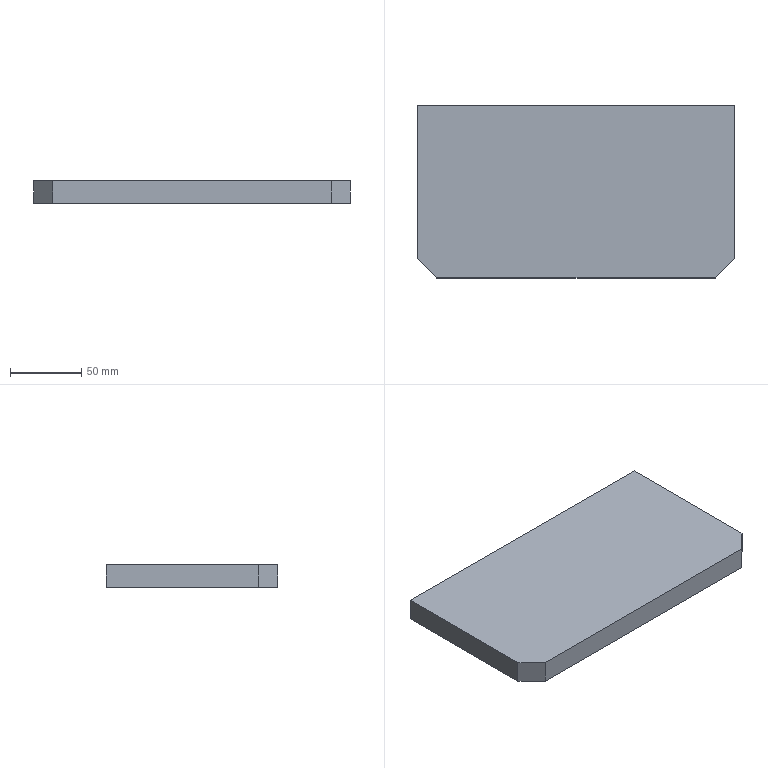Component | SolidWorks | WeldedI-beam-1_250I-beamStiffener-1 | 1 solid | 8 faces | box 222 x 120.5 x 16 mm | volume 425100 mm3 | plane 8 | material Plain Carbon Steel
STEP:
#1=COLOUR_RGB('',0.7922,0.8196,0.9333);
#2=FILL_AREA_STYLE_COLOUR('',#1);
#3=FILL_AREA_STYLE('',(#2));
#4=SURFACE_STYLE_FILL_AREA(#3);
#5=SURFACE_SIDE_STYLE('',(#4));
#6=SURFACE_STYLE_USAGE(.BOTH.,#5);
#7=PRESENTATION_STYLE_ASSIGNMENT((#6));
#8=CARTESIAN_POINT('',(-255.255,115.423,245.041));
#9=VERTEX_POINT('',#8);
#10=CARTESIAN_POINT('',(-255.255,111.21,245.041));
#11=VERTEX_POINT('',#10);
#12=CARTESIAN_POINT('',(-255.255,115.423,245.041));
#13=DIRECTION('',(0.,-1.,-0.));
#14=VECTOR('',#13,39.37);
#15=LINE('',#12,#14);
#16=EDGE_CURVE('',#9,#11,#15,.T.);
#17=ORIENTED_EDGE('',*,*,#16,.F.);
#18=CARTESIAN_POINT('',(-255.255,115.423,244.411));
#19=VERTEX_POINT('',#18);
#20=CARTESIAN_POINT('',(-255.255,115.423,244.411));
#21=DIRECTION('',(0.,-0.,1.));
#22=VECTOR('',#21,39.37);
#23=LINE('',#20,#22);
#24=EDGE_CURVE('',#19,#9,#23,.T.);
#25=ORIENTED_EDGE('',*,*,#24,.F.);
#26=CARTESIAN_POINT('',(-255.255,111.21,244.411));
#27=VERTEX_POINT('',#26);
#28=CARTESIAN_POINT('',(-255.255,115.423,244.411));
#29=DIRECTION('',(0.,-1.,-0.));
#30=VECTOR('',#29,39.37);
#31=LINE('',#28,#30);
#32=EDGE_CURVE('',#19,#27,#31,.T.);
#33=ORIENTED_EDGE('',*,*,#32,.T.);
#34=CARTESIAN_POINT('',(-255.255,111.21,244.411));
#35=DIRECTION('',(0.,-0.,1.));
#36=VECTOR('',#35,39.37);
#37=LINE('',#34,#36);
#38=EDGE_CURVE('',#27,#11,#37,.T.);
#39=ORIENTED_EDGE('',*,*,#38,.T.);
#40=EDGE_LOOP('',(#17,#25,#33,#39));
#41=FACE_OUTER_BOUND('',#40,.T.);
#42=CARTESIAN_POINT('',(-255.255,115.423,244.411));
#43=DIRECTION('',(-1.,-0.,-0.));
#44=DIRECTION('',(0.,-1.,-0.));
#45=AXIS2_PLACEMENT_3D('',#42,#43,#44);
#46=PLANE('',#45);
#47=ADVANCED_FACE('',(#41),#46,.T.);
#48=CARTESIAN_POINT('',(-246.514,115.423,245.041));
#49=VERTEX_POINT('',#48);
#50=CARTESIAN_POINT('',(-255.255,115.423,245.041));
#51=DIRECTION('',(-1.,0.,0.));
#52=VECTOR('',#51,39.37);
#53=LINE('',#50,#52);
#54=EDGE_CURVE('',#49,#9,#53,.T.);
#55=ORIENTED_EDGE('',*,*,#54,.F.);
#56=CARTESIAN_POINT('',(-246.514,115.423,244.411));
#57=VERTEX_POINT('',#56);
#58=CARTESIAN_POINT('',(-246.514,115.423,244.411));
#59=DIRECTION('',(0.,-0.,1.));
#60=VECTOR('',#59,39.37);
#61=LINE('',#58,#60);
#62=EDGE_CURVE('',#57,#49,#61,.T.);
#63=ORIENTED_EDGE('',*,*,#62,.F.);
#64=CARTESIAN_POINT('',(-255.255,115.423,244.411));
#65=DIRECTION('',(-1.,0.,0.));
#66=VECTOR('',#65,39.37);
#67=LINE('',#64,#66);
#68=EDGE_CURVE('',#57,#19,#67,.T.);
#69=ORIENTED_EDGE('',*,*,#68,.T.);
#70=ORIENTED_EDGE('',*,*,#24,.T.);
#71=EDGE_LOOP('',(#55,#63,#69,#70));
#72=FACE_OUTER_BOUND('',#71,.T.);
#73=CARTESIAN_POINT('',(-255.255,115.423,244.411));
#74=DIRECTION('',(0.,1.,0.));
#75=DIRECTION('',(-1.,0.,0.));
#76=AXIS2_PLACEMENT_3D('',#73,#74,#75);
#77=PLANE('',#76);
#78=ADVANCED_FACE('',(#72),#77,.T.);
#79=CARTESIAN_POINT('',(-246.514,111.21,245.041));
#80=VERTEX_POINT('',#79);
#81=CARTESIAN_POINT('',(-246.514,115.423,245.041));
#82=DIRECTION('',(0.,1.,0.));
#83=VECTOR('',#82,39.37);
#84=LINE('',#81,#83);
#85=EDGE_CURVE('',#80,#49,#84,.T.);
#86=ORIENTED_EDGE('',*,*,#85,.F.);
#87=CARTESIAN_POINT('',(-246.514,111.21,244.411));
#88=VERTEX_POINT('',#87);
#89=CARTESIAN_POINT('',(-246.514,111.21,244.411));
#90=DIRECTION('',(0.,-0.,1.));
#91=VECTOR('',#90,39.37);
#92=LINE('',#89,#91);
#93=EDGE_CURVE('',#88,#80,#92,.T.);
#94=ORIENTED_EDGE('',*,*,#93,.F.);
#95=CARTESIAN_POINT('',(-246.514,115.423,244.411));
#96=DIRECTION('',(0.,1.,0.));
#97=VECTOR('',#96,39.37);
#98=LINE('',#95,#97);
#99=EDGE_CURVE('',#88,#57,#98,.T.);
#100=ORIENTED_EDGE('',*,*,#99,.T.);
#101=ORIENTED_EDGE('',*,*,#62,.T.);
#102=EDGE_LOOP('',(#86,#94,#100,#101));
#103=FACE_OUTER_BOUND('',#102,.T.);
#104=CARTESIAN_POINT('',(-246.514,115.423,244.411));
#105=DIRECTION('',(1.,-0.,-0.));
#106=DIRECTION('',(0.,1.,0.));
#107=AXIS2_PLACEMENT_3D('',#104,#105,#106);
#108=PLANE('',#107);
#109=ADVANCED_FACE('',(#103),#108,.T.);
#110=CARTESIAN_POINT('',(-247.046,110.678,245.041));
#111=VERTEX_POINT('',#110);
#112=CARTESIAN_POINT('',(-247.046,110.678,245.041));
#113=DIRECTION('',(0.7071,0.7071,0.));
#114=VECTOR('',#113,39.37);
#115=LINE('',#112,#114);
#116=EDGE_CURVE('',#111,#80,#115,.T.);
#117=ORIENTED_EDGE('',*,*,#116,.F.);
#118=CARTESIAN_POINT('',(-247.046,110.678,244.411));
#119=VERTEX_POINT('',#118);
#120=CARTESIAN_POINT('',(-247.046,110.678,244.411));
#121=DIRECTION('',(0.,-0.,1.));
#122=VECTOR('',#121,39.37);
#123=LINE('',#120,#122);
#124=EDGE_CURVE('',#119,#111,#123,.T.);
#125=ORIENTED_EDGE('',*,*,#124,.F.);
#126=CARTESIAN_POINT('',(-247.046,110.678,244.411));
#127=DIRECTION('',(0.7071,0.7071,0.));
#128=VECTOR('',#127,39.37);
#129=LINE('',#126,#128);
#130=EDGE_CURVE('',#119,#88,#129,.T.);
#131=ORIENTED_EDGE('',*,*,#130,.T.);
#132=ORIENTED_EDGE('',*,*,#93,.T.);
#133=EDGE_LOOP('',(#117,#125,#131,#132));
#134=FACE_OUTER_BOUND('',#133,.T.);
#135=CARTESIAN_POINT('',(-247.046,110.678,244.411));
#136=DIRECTION('',(0.7071,-0.7071,-0.));
#137=DIRECTION('',(0.7071,0.7071,0.));
#138=AXIS2_PLACEMENT_3D('',#135,#136,#137);
#139=PLANE('',#138);
#140=ADVANCED_FACE('',(#134),#139,.T.);
#141=CARTESIAN_POINT('',(-254.723,110.678,245.041));
#142=VERTEX_POINT('',#141);
#143=CARTESIAN_POINT('',(-254.723,110.678,245.041));
#144=DIRECTION('',(1.,0.,0.));
#145=VECTOR('',#144,39.37);
#146=LINE('',#143,#145);
#147=EDGE_CURVE('',#142,#111,#146,.T.);
#148=ORIENTED_EDGE('',*,*,#147,.F.);
#149=CARTESIAN_POINT('',(-254.723,110.678,244.411));
#150=VERTEX_POINT('',#149);
#151=CARTESIAN_POINT('',(-254.723,110.678,244.411));
#152=DIRECTION('',(0.,-0.,1.));
#153=VECTOR('',#152,39.37);
#154=LINE('',#151,#153);
#155=EDGE_CURVE('',#150,#142,#154,.T.);
#156=ORIENTED_EDGE('',*,*,#155,.F.);
#157=CARTESIAN_POINT('',(-254.723,110.678,244.411));
#158=DIRECTION('',(1.,0.,0.));
#159=VECTOR('',#158,39.37);
#160=LINE('',#157,#159);
#161=EDGE_CURVE('',#150,#119,#160,.T.);
#162=ORIENTED_EDGE('',*,*,#161,.T.);
#163=ORIENTED_EDGE('',*,*,#124,.T.);
#164=EDGE_LOOP('',(#148,#156,#162,#163));
#165=FACE_OUTER_BOUND('',#164,.T.);
#166=CARTESIAN_POINT('',(-254.723,110.678,244.411));
#167=DIRECTION('',(0.,-1.,-0.));
#168=DIRECTION('',(1.,0.,0.));
#169=AXIS2_PLACEMENT_3D('',#166,#167,#168);
#170=PLANE('',#169);
#171=ADVANCED_FACE('',(#165),#170,.T.);
#172=CARTESIAN_POINT('',(-255.255,111.21,245.041));
#173=DIRECTION('',(0.7071,-0.7071,-0.));
#174=VECTOR('',#173,39.37);
#175=LINE('',#172,#174);
#176=EDGE_CURVE('',#11,#142,#175,.T.);
#177=ORIENTED_EDGE('',*,*,#176,.F.);
#178=ORIENTED_EDGE('',*,*,#38,.F.);
#179=CARTESIAN_POINT('',(-255.255,111.21,244.411));
#180=DIRECTION('',(0.7071,-0.7071,-0.));
#181=VECTOR('',#180,39.37);
#182=LINE('',#179,#181);
#183=EDGE_CURVE('',#27,#150,#182,.T.);
#184=ORIENTED_EDGE('',*,*,#183,.T.);
#185=ORIENTED_EDGE('',*,*,#155,.T.);
#186=EDGE_LOOP('',(#177,#178,#184,#185));
#187=FACE_OUTER_BOUND('',#186,.T.);
#188=CARTESIAN_POINT('',(-255.255,111.21,244.411));
#189=DIRECTION('',(-0.7071,-0.7071,-0.));
#190=DIRECTION('',(0.7071,-0.7071,-0.));
#191=AXIS2_PLACEMENT_3D('',#188,#189,#190);
#192=PLANE('',#191);
#193=ADVANCED_FACE('',(#187),#192,.T.);
#194=ORIENTED_EDGE('',*,*,#32,.F.);
#195=ORIENTED_EDGE('',*,*,#68,.F.);
#196=ORIENTED_EDGE('',*,*,#99,.F.);
#197=ORIENTED_EDGE('',*,*,#130,.F.);
#198=ORIENTED_EDGE('',*,*,#161,.F.);
#199=ORIENTED_EDGE('',*,*,#183,.F.);
#200=EDGE_LOOP('',(#194,#195,#196,#197,#198,#199));
#201=FACE_OUTER_BOUND('',#200,.T.);
#202=CARTESIAN_POINT('',(-255.255,115.423,244.411));
#203=DIRECTION('',(0.,-0.,1.));
#204=DIRECTION('',(0.,-1.,-0.));
#205=AXIS2_PLACEMENT_3D('',#202,#203,#204);
#206=PLANE('',#205);
#207=ADVANCED_FACE('',(#201),#206,.F.);
#208=ORIENTED_EDGE('',*,*,#16,.T.);
#209=ORIENTED_EDGE('',*,*,#176,.T.);
#210=ORIENTED_EDGE('',*,*,#147,.T.);
#211=ORIENTED_EDGE('',*,*,#116,.T.);
#212=ORIENTED_EDGE('',*,*,#85,.T.);
#213=ORIENTED_EDGE('',*,*,#54,.T.);
#214=EDGE_LOOP('',(#208,#209,#210,#211,#212,#213));
#215=FACE_OUTER_BOUND('',#214,.T.);
#216=CARTESIAN_POINT('',(-255.255,115.423,245.041));
#217=DIRECTION('',(0.,-0.,1.));
#218=DIRECTION('',(0.,-1.,-0.));
#219=AXIS2_PLACEMENT_3D('',#216,#217,#218);
#220=PLANE('',#219);
#221=ADVANCED_FACE('',(#215),#220,.T.);
#222=CLOSED_SHELL('',(#47,#78,#109,#140,#171,#193,#207,#221));
#223=MANIFOLD_SOLID_BREP('',#222);
#224=STYLED_ITEM('',(#7),#223);
#225=PRESENTATION_LAYER_ASSIGNMENT('','',(#224));
#226=(LENGTH_UNIT()NAMED_UNIT(*)SI_UNIT($,.METRE.));
#227=LENGTH_MEASURE_WITH_UNIT(LENGTH_MEASURE(0.0254),#226);
#228=DIMENSIONAL_EXPONENTS(1.,0.,0.,0.,0.,0.,0.);
#229=(CONVERSION_BASED_UNIT('',#227)LENGTH_UNIT()NAMED_UNIT(#228));
#230=UNCERTAINTY_MEASURE_WITH_UNIT(LENGTH_MEASURE(0.00001),#229,'','');
#231=(NAMED_UNIT(*)PLANE_ANGLE_UNIT()SI_UNIT($,.RADIAN.));
#232=(NAMED_UNIT(*)SI_UNIT($,.STERADIAN.)SOLID_ANGLE_UNIT());
#233=(GEOMETRIC_REPRESENTATION_CONTEXT(3)GLOBAL_UNCERTAINTY_ASSIGNED_CONTEXT((#230))GLOBAL_UNIT_ASSIGNED_CONTEXT((#229,#231,#232))REPRESENTATION_CONTEXT('',''));
#234=MECHANICAL_DESIGN_GEOMETRIC_PRESENTATION_REPRESENTATION('',(#224),#233);
#235=CARTESIAN_POINT('',(0.,0.,0.));
#236=DIRECTION('',(0.,0.,1.));
#237=DIRECTION('',(1.,0.,0.));
#238=AXIS2_PLACEMENT_3D('',#235,#236,#237);
#239=(LENGTH_UNIT()NAMED_UNIT(*)SI_UNIT($,.METRE.));
#240=LENGTH_MEASURE_WITH_UNIT(LENGTH_MEASURE(0.0254),#239);
#241=DIMENSIONAL_EXPONENTS(1.,0.,0.,0.,0.,0.,0.);
#242=(CONVERSION_BASED_UNIT('',#240)LENGTH_UNIT()NAMED_UNIT(#241));
#243=UNCERTAINTY_MEASURE_WITH_UNIT(LENGTH_MEASURE(0.00001),#242,'','');
#244=(NAMED_UNIT(*)PLANE_ANGLE_UNIT()SI_UNIT($,.RADIAN.));
#245=(NAMED_UNIT(*)SI_UNIT($,.STERADIAN.)SOLID_ANGLE_UNIT());
#246=(GEOMETRIC_REPRESENTATION_CONTEXT(3)GLOBAL_UNCERTAINTY_ASSIGNED_CONTEXT((#243))GLOBAL_UNIT_ASSIGNED_CONTEXT((#242,#244,#245))REPRESENTATION_CONTEXT('',''));
#247=ADVANCED_BREP_SHAPE_REPRESENTATION('',(#223,#238),#246);